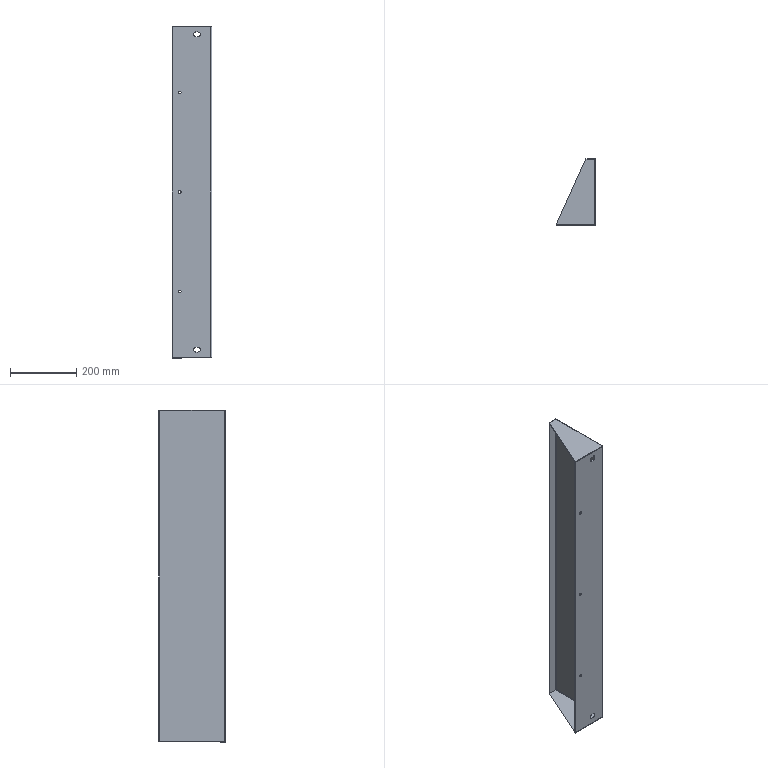Component | SolidWorks | Brow-1 | 1 solid | 54 faces | volume 559424 mm3 | plane 26 | cylinder 20 | spline 8 | commonest cylinder face diameters 8 x6 14 x6 3 x4 6 x4